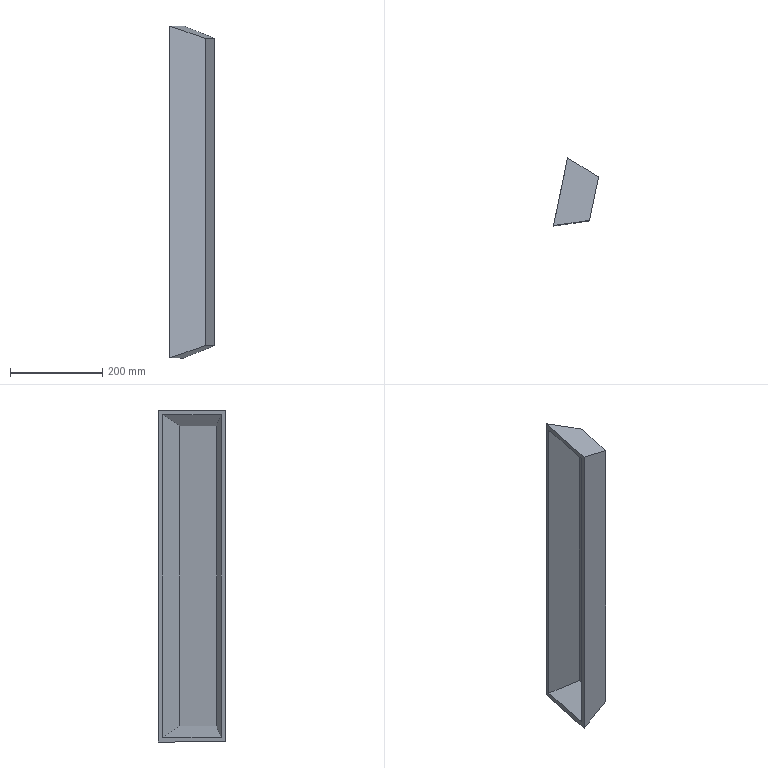Component | SolidWorks | AluminumIngotContainer-10 | 1 solid | 11 faces | box 97.54 x 146.85 x 720 mm | volume 1760907 mm3 | plane 11
build123d program:
from build123d import *

# Parameters (mm, degrees)
SKETCH1_W           = 150
SKETCH1_H           = 720
BOSS_EXTRUDE1_DEPTH = 74
BOSS_EXTRUDE1_TAPER = 20
SHELL1_T            = -10


with BuildPart() as part:
    # Sketch1 → Boss-Extrude1 (new body)
    with BuildSketch(Plane.XY):
        Rectangle(SKETCH1_W, SKETCH1_H)
    extrude(amount=BOSS_EXTRUDE1_DEPTH, taper=BOSS_EXTRUDE1_TAPER)

    # Shell1
    shell1_openings = [part.faces().sort_by_distance(p)[0] for p in [
        (0, 0, 0),
    ]]
    offset(amount=SHELL1_T, openings=shell1_openings, kind=Kind.INTERSECTION)


solid = part.part

# Placed as in the assembly
solid = solid.moved(Location((746.968, 361.921, 495), (90, 78.234, -180)))
STEP:
#1=COLOUR_RGB('',0.7922,0.8196,0.9333);
#2=FILL_AREA_STYLE_COLOUR('',#1);
#3=FILL_AREA_STYLE('',(#2));
#4=SURFACE_STYLE_FILL_AREA(#3);
#5=SURFACE_SIDE_STYLE('',(#4));
#6=SURFACE_STYLE_USAGE(.BOTH.,#5);
#7=PRESENTATION_STYLE_ASSIGNMENT((#6));
#8=CARTESIAN_POINT('',(30.01,17.14,5.315));
#9=VERTEX_POINT('',#8);
#10=CARTESIAN_POINT('',(30.01,17.14,33.661));
#11=VERTEX_POINT('',#10);
#12=CARTESIAN_POINT('',(30.01,17.14,5.315));
#13=DIRECTION('',(0.,0.,1.));
#14=VECTOR('',#13,39.37);
#15=LINE('',#12,#14);
#16=EDGE_CURVE('',#9,#11,#15,.T.);
#17=ORIENTED_EDGE('',*,*,#16,.F.);
#18=CARTESIAN_POINT('',(28.806,11.358,5.315));
#19=VERTEX_POINT('',#18);
#20=CARTESIAN_POINT('',(28.806,11.358,5.315));
#21=DIRECTION('',(0.2039,0.979,-0.));
#22=VECTOR('',#21,39.37);
#23=LINE('',#20,#22);
#24=EDGE_CURVE('',#19,#9,#23,.T.);
#25=ORIENTED_EDGE('',*,*,#24,.F.);
#26=CARTESIAN_POINT('',(28.806,11.358,33.661));
#27=VERTEX_POINT('',#26);
#28=CARTESIAN_POINT('',(28.806,11.358,5.315));
#29=DIRECTION('',(-0.,-0.,-1.));
#30=VECTOR('',#29,39.37);
#31=LINE('',#28,#30);
#32=EDGE_CURVE('',#27,#19,#31,.T.);
#33=ORIENTED_EDGE('',*,*,#32,.F.);
#34=CARTESIAN_POINT('',(28.806,11.358,33.661));
#35=DIRECTION('',(-0.2039,-0.979,0.));
#36=VECTOR('',#35,39.37);
#37=LINE('',#34,#36);
#38=EDGE_CURVE('',#11,#27,#37,.T.);
#39=ORIENTED_EDGE('',*,*,#38,.F.);
#40=EDGE_LOOP('',(#17,#25,#33,#39));
#41=FACE_OUTER_BOUND('',#40,.T.);
#42=CARTESIAN_POINT('',(28.892,11.768,5.734));
#43=VERTEX_POINT('',#42);
#44=CARTESIAN_POINT('',(29.925,16.729,5.734));
#45=VERTEX_POINT('',#44);
#46=CARTESIAN_POINT('',(29.408,14.249,5.734));
#47=DIRECTION('',(0.2039,0.979,-0.));
#48=VECTOR('',#47,39.37);
#49=LINE('',#46,#48);
#50=EDGE_CURVE('',#43,#45,#49,.T.);
#51=ORIENTED_EDGE('',*,*,#50,.T.);
#52=CARTESIAN_POINT('',(29.925,16.729,33.242));
#53=VERTEX_POINT('',#52);
#54=CARTESIAN_POINT('',(29.925,16.729,19.488));
#55=DIRECTION('',(0.,0.,1.));
#56=VECTOR('',#55,39.37);
#57=LINE('',#54,#56);
#58=EDGE_CURVE('',#45,#53,#57,.T.);
#59=ORIENTED_EDGE('',*,*,#58,.T.);
#60=CARTESIAN_POINT('',(28.892,11.768,33.242));
#61=VERTEX_POINT('',#60);
#62=CARTESIAN_POINT('',(29.408,14.249,33.242));
#63=DIRECTION('',(-0.2039,-0.979,0.));
#64=VECTOR('',#63,39.37);
#65=LINE('',#62,#64);
#66=EDGE_CURVE('',#53,#61,#65,.T.);
#67=ORIENTED_EDGE('',*,*,#66,.T.);
#68=CARTESIAN_POINT('',(28.892,11.768,19.488));
#69=DIRECTION('',(-0.,-0.,-1.));
#70=VECTOR('',#69,39.37);
#71=LINE('',#68,#70);
#72=EDGE_CURVE('',#61,#43,#71,.T.);
#73=ORIENTED_EDGE('',*,*,#72,.T.);
#74=EDGE_LOOP('',(#51,#59,#67,#73));
#75=FACE_BOUND('',#74,.T.);
#76=CARTESIAN_POINT('',(29.408,14.249,19.488));
#77=DIRECTION('',(-0.979,0.2039,0.));
#78=DIRECTION('',(0.2039,0.979,-0.));
#79=AXIS2_PLACEMENT_3D('',#76,#77,#78);
#80=PLANE('',#79);
#81=ADVANCED_FACE('',(#41,#75),#80,.T.);
#82=ORIENTED_EDGE('',*,*,#16,.T.);
#83=CARTESIAN_POINT('',(32.646,15.507,32.601));
#84=VERTEX_POINT('',#83);
#85=CARTESIAN_POINT('',(31.548,16.188,33.043));
#86=DIRECTION('',(-0.8045,0.4981,0.3236));
#87=VECTOR('',#86,39.37);
#88=LINE('',#85,#87);
#89=EDGE_CURVE('',#84,#11,#88,.T.);
#90=ORIENTED_EDGE('',*,*,#89,.F.);
#91=CARTESIAN_POINT('',(32.646,15.507,6.375));
#92=VERTEX_POINT('',#91);
#93=CARTESIAN_POINT('',(32.646,15.507,19.488));
#94=DIRECTION('',(0.,0.,1.));
#95=VECTOR('',#94,39.37);
#96=LINE('',#93,#95);
#97=EDGE_CURVE('',#92,#84,#96,.T.);
#98=ORIENTED_EDGE('',*,*,#97,.F.);
#99=CARTESIAN_POINT('',(30.01,17.14,5.315));
#100=DIRECTION('',(-0.8045,0.4981,-0.3236));
#101=VECTOR('',#100,39.37);
#102=LINE('',#99,#101);
#103=EDGE_CURVE('',#92,#9,#102,.T.);
#104=ORIENTED_EDGE('',*,*,#103,.T.);
#105=EDGE_LOOP('',(#82,#90,#98,#104));
#106=FACE_OUTER_BOUND('',#105,.T.);
#107=CARTESIAN_POINT('',(30.01,17.14,5.315));
#108=DIRECTION('',(0.5264,0.8502,-0.));
#109=DIRECTION('',(0.8502,-0.5264,-0.));
#110=AXIS2_PLACEMENT_3D('',#107,#108,#109);
#111=PLANE('',#110);
#112=ADVANCED_FACE('',(#106),#111,.T.);
#113=ORIENTED_EDGE('',*,*,#38,.T.);
#114=CARTESIAN_POINT('',(31.874,11.802,32.601));
#115=VERTEX_POINT('',#114);
#116=CARTESIAN_POINT('',(37.396,12.601,30.693));
#117=DIRECTION('',(-0.9364,-0.1355,0.3236));
#118=VECTOR('',#117,39.37);
#119=LINE('',#116,#118);
#120=EDGE_CURVE('',#115,#27,#119,.T.);
#121=ORIENTED_EDGE('',*,*,#120,.F.);
#122=CARTESIAN_POINT('',(32.26,13.655,32.601));
#123=DIRECTION('',(-0.2039,-0.979,0.));
#124=VECTOR('',#123,39.37);
#125=LINE('',#122,#124);
#126=EDGE_CURVE('',#84,#115,#125,.T.);
#127=ORIENTED_EDGE('',*,*,#126,.F.);
#128=ORIENTED_EDGE('',*,*,#89,.T.);
#129=EDGE_LOOP('',(#113,#121,#127,#128));
#130=FACE_OUTER_BOUND('',#129,.T.);
#131=CARTESIAN_POINT('',(28.806,11.358,33.661));
#132=DIRECTION('',(0.3348,-0.06974,0.9397));
#133=DIRECTION('',(-0.9199,0.1916,0.342));
#134=AXIS2_PLACEMENT_3D('',#131,#132,#133);
#135=PLANE('',#134);
#136=ADVANCED_FACE('',(#130),#135,.T.);
#137=ORIENTED_EDGE('',*,*,#32,.T.);
#138=CARTESIAN_POINT('',(31.874,11.802,6.375));
#139=VERTEX_POINT('',#138);
#140=CARTESIAN_POINT('',(28.806,11.358,5.315));
#141=DIRECTION('',(-0.9364,-0.1355,-0.3236));
#142=VECTOR('',#141,39.37);
#143=LINE('',#140,#142);
#144=EDGE_CURVE('',#139,#19,#143,.T.);
#145=ORIENTED_EDGE('',*,*,#144,.F.);
#146=CARTESIAN_POINT('',(31.874,11.802,19.488));
#147=DIRECTION('',(-0.,-0.,-1.));
#148=VECTOR('',#147,39.37);
#149=LINE('',#146,#148);
#150=EDGE_CURVE('',#115,#139,#149,.T.);
#151=ORIENTED_EDGE('',*,*,#150,.F.);
#152=ORIENTED_EDGE('',*,*,#120,.T.);
#153=EDGE_LOOP('',(#137,#145,#151,#152));
#154=FACE_OUTER_BOUND('',#153,.T.);
#155=CARTESIAN_POINT('',(28.806,11.358,5.315));
#156=DIRECTION('',(0.1432,-0.9897,0.));
#157=DIRECTION('',(-0.9897,-0.1432,0.));
#158=AXIS2_PLACEMENT_3D('',#155,#156,#157);
#159=PLANE('',#158);
#160=ADVANCED_FACE('',(#154),#159,.T.);
#161=ORIENTED_EDGE('',*,*,#24,.T.);
#162=ORIENTED_EDGE('',*,*,#103,.F.);
#163=CARTESIAN_POINT('',(32.26,13.655,6.375));
#164=DIRECTION('',(0.2039,0.979,-0.));
#165=VECTOR('',#164,39.37);
#166=LINE('',#163,#165);
#167=EDGE_CURVE('',#139,#92,#166,.T.);
#168=ORIENTED_EDGE('',*,*,#167,.F.);
#169=ORIENTED_EDGE('',*,*,#144,.T.);
#170=EDGE_LOOP('',(#161,#162,#168,#169));
#171=FACE_OUTER_BOUND('',#170,.T.);
#172=CARTESIAN_POINT('',(28.806,11.358,5.315));
#173=DIRECTION('',(0.3348,-0.06974,-0.9397));
#174=DIRECTION('',(0.9199,-0.1916,0.342));
#175=AXIS2_PLACEMENT_3D('',#172,#173,#174);
#176=PLANE('',#175);
#177=ADVANCED_FACE('',(#171),#176,.T.);
#178=ORIENTED_EDGE('',*,*,#97,.T.);
#179=ORIENTED_EDGE('',*,*,#126,.T.);
#180=ORIENTED_EDGE('',*,*,#150,.T.);
#181=ORIENTED_EDGE('',*,*,#167,.T.);
#182=EDGE_LOOP('',(#178,#179,#180,#181));
#183=FACE_OUTER_BOUND('',#182,.T.);
#184=CARTESIAN_POINT('',(32.26,13.655,19.488));
#185=DIRECTION('',(-0.979,0.2039,0.));
#186=DIRECTION('',(0.2039,0.979,-0.));
#187=AXIS2_PLACEMENT_3D('',#184,#185,#186);
#188=PLANE('',#187);
#189=ADVANCED_FACE('',(#183),#188,.F.);
#190=ORIENTED_EDGE('',*,*,#58,.F.);
#191=CARTESIAN_POINT('',(32.205,15.318,6.651));
#192=VERTEX_POINT('',#191);
#193=CARTESIAN_POINT('',(29.707,16.864,5.646));
#194=DIRECTION('',(-0.8045,0.4981,-0.3236));
#195=VECTOR('',#194,39.37);
#196=LINE('',#193,#195);
#197=EDGE_CURVE('',#192,#45,#196,.T.);
#198=ORIENTED_EDGE('',*,*,#197,.F.);
#199=CARTESIAN_POINT('',(32.205,15.318,32.325));
#200=VERTEX_POINT('',#199);
#201=CARTESIAN_POINT('',(32.205,15.318,19.488));
#202=DIRECTION('',(0.,0.,1.));
#203=VECTOR('',#202,39.37);
#204=LINE('',#201,#203);
#205=EDGE_CURVE('',#192,#200,#204,.T.);
#206=ORIENTED_EDGE('',*,*,#205,.T.);
#207=CARTESIAN_POINT('',(31.244,15.913,32.712));
#208=DIRECTION('',(-0.8045,0.4981,0.3236));
#209=VECTOR('',#208,39.37);
#210=LINE('',#207,#209);
#211=EDGE_CURVE('',#200,#53,#210,.T.);
#212=ORIENTED_EDGE('',*,*,#211,.T.);
#213=EDGE_LOOP('',(#190,#198,#206,#212));
#214=FACE_OUTER_BOUND('',#213,.T.);
#215=CARTESIAN_POINT('',(29.803,16.805,5.315));
#216=DIRECTION('',(0.5264,0.8502,-0.));
#217=DIRECTION('',(0.8502,-0.5264,-0.));
#218=AXIS2_PLACEMENT_3D('',#215,#216,#217);
#219=PLANE('',#218);
#220=ADVANCED_FACE('',(#214),#219,.F.);
#221=ORIENTED_EDGE('',*,*,#66,.F.);
#222=ORIENTED_EDGE('',*,*,#211,.F.);
#223=CARTESIAN_POINT('',(31.545,12.152,32.325));
#224=VERTEX_POINT('',#223);
#225=CARTESIAN_POINT('',(31.875,13.735,32.325));
#226=DIRECTION('',(-0.2039,-0.979,0.));
#227=VECTOR('',#226,39.37);
#228=LINE('',#225,#227);
#229=EDGE_CURVE('',#200,#224,#228,.T.);
#230=ORIENTED_EDGE('',*,*,#229,.T.);
#231=CARTESIAN_POINT('',(37.228,12.975,30.362));
#232=DIRECTION('',(-0.9364,-0.1355,0.3236));
#233=VECTOR('',#232,39.37);
#234=LINE('',#231,#233);
#235=EDGE_CURVE('',#224,#61,#234,.T.);
#236=ORIENTED_EDGE('',*,*,#235,.T.);
#237=EDGE_LOOP('',(#221,#222,#230,#236));
#238=FACE_OUTER_BOUND('',#237,.T.);
#239=CARTESIAN_POINT('',(28.674,11.386,33.291));
#240=DIRECTION('',(0.3348,-0.06974,0.9397));
#241=DIRECTION('',(-0.9199,0.1916,0.342));
#242=AXIS2_PLACEMENT_3D('',#239,#240,#241);
#243=PLANE('',#242);
#244=ADVANCED_FACE('',(#238),#243,.F.);
#245=ORIENTED_EDGE('',*,*,#72,.F.);
#246=ORIENTED_EDGE('',*,*,#235,.F.);
#247=CARTESIAN_POINT('',(31.545,12.152,6.651));
#248=VERTEX_POINT('',#247);
#249=CARTESIAN_POINT('',(31.545,12.152,19.488));
#250=DIRECTION('',(-0.,-0.,-1.));
#251=VECTOR('',#250,39.37);
#252=LINE('',#249,#251);
#253=EDGE_CURVE('',#224,#248,#252,.T.);
#254=ORIENTED_EDGE('',*,*,#253,.T.);
#255=CARTESIAN_POINT('',(28.638,11.732,5.646));
#256=DIRECTION('',(-0.9364,-0.1355,-0.3236));
#257=VECTOR('',#256,39.37);
#258=LINE('',#255,#257);
#259=EDGE_CURVE('',#248,#43,#258,.T.);
#260=ORIENTED_EDGE('',*,*,#259,.T.);
#261=EDGE_LOOP('',(#245,#246,#254,#260));
#262=FACE_OUTER_BOUND('',#261,.T.);
#263=CARTESIAN_POINT('',(28.75,11.748,5.315));
#264=DIRECTION('',(0.1432,-0.9897,0.));
#265=DIRECTION('',(-0.9897,-0.1432,0.));
#266=AXIS2_PLACEMENT_3D('',#263,#264,#265);
#267=PLANE('',#266);
#268=ADVANCED_FACE('',(#262),#267,.F.);
#269=ORIENTED_EDGE('',*,*,#50,.F.);
#270=ORIENTED_EDGE('',*,*,#259,.F.);
#271=CARTESIAN_POINT('',(31.875,13.735,6.651));
#272=DIRECTION('',(0.2039,0.979,-0.));
#273=VECTOR('',#272,39.37);
#274=LINE('',#271,#273);
#275=EDGE_CURVE('',#248,#192,#274,.T.);
#276=ORIENTED_EDGE('',*,*,#275,.T.);
#277=ORIENTED_EDGE('',*,*,#197,.T.);
#278=EDGE_LOOP('',(#269,#270,#276,#277));
#279=FACE_OUTER_BOUND('',#278,.T.);
#280=CARTESIAN_POINT('',(28.674,11.386,5.685));
#281=DIRECTION('',(0.3348,-0.06974,-0.9397));
#282=DIRECTION('',(0.9199,-0.1916,0.342));
#283=AXIS2_PLACEMENT_3D('',#280,#281,#282);
#284=PLANE('',#283);
#285=ADVANCED_FACE('',(#279),#284,.F.);
#286=ORIENTED_EDGE('',*,*,#205,.F.);
#287=ORIENTED_EDGE('',*,*,#275,.F.);
#288=ORIENTED_EDGE('',*,*,#253,.F.);
#289=ORIENTED_EDGE('',*,*,#229,.F.);
#290=EDGE_LOOP('',(#286,#287,#288,#289));
#291=FACE_OUTER_BOUND('',#290,.T.);
#292=CARTESIAN_POINT('',(31.875,13.735,19.488));
#293=DIRECTION('',(-0.979,0.2039,0.));
#294=DIRECTION('',(0.2039,0.979,-0.));
#295=AXIS2_PLACEMENT_3D('',#292,#293,#294);
#296=PLANE('',#295);
#297=ADVANCED_FACE('',(#291),#296,.T.);
#298=CLOSED_SHELL('',(#81,#112,#136,#160,#177,#189,#220,#244,#268,#285,#297));
#299=MANIFOLD_SOLID_BREP('',#298);
#300=STYLED_ITEM('',(#7),#299);
#301=(LENGTH_UNIT()NAMED_UNIT(*)SI_UNIT($,.METRE.));
#302=LENGTH_MEASURE_WITH_UNIT(LENGTH_MEASURE(0.0254),#301);
#303=DIMENSIONAL_EXPONENTS(1.,0.,0.,0.,0.,0.,0.);
#304=(CONVERSION_BASED_UNIT('',#302)LENGTH_UNIT()NAMED_UNIT(#303));
#305=UNCERTAINTY_MEASURE_WITH_UNIT(LENGTH_MEASURE(0.00001),#304,'','');
#306=(NAMED_UNIT(*)PLANE_ANGLE_UNIT()SI_UNIT($,.RADIAN.));
#307=(NAMED_UNIT(*)SI_UNIT($,.STERADIAN.)SOLID_ANGLE_UNIT());
#308=(GEOMETRIC_REPRESENTATION_CONTEXT(3)GLOBAL_UNCERTAINTY_ASSIGNED_CONTEXT((#305))GLOBAL_UNIT_ASSIGNED_CONTEXT((#304,#306,#307))REPRESENTATION_CONTEXT('',''));
#309=MECHANICAL_DESIGN_GEOMETRIC_PRESENTATION_REPRESENTATION('',(#300),#308);
#310=PRESENTATION_LAYER_ASSIGNMENT('','',(#300));
#311=CARTESIAN_POINT('',(0.,0.,0.));
#312=DIRECTION('',(0.,0.,1.));
#313=DIRECTION('',(1.,0.,0.));
#314=AXIS2_PLACEMENT_3D('',#311,#312,#313);
#315=(LENGTH_UNIT()NAMED_UNIT(*)SI_UNIT($,.METRE.));
#316=LENGTH_MEASURE_WITH_UNIT(LENGTH_MEASURE(0.0254),#315);
#317=DIMENSIONAL_EXPONENTS(1.,0.,0.,0.,0.,0.,0.);
#318=(CONVERSION_BASED_UNIT('',#316)LENGTH_UNIT()NAMED_UNIT(#317));
#319=UNCERTAINTY_MEASURE_WITH_UNIT(LENGTH_MEASURE(0.00001),#318,'','');
#320=(NAMED_UNIT(*)PLANE_ANGLE_UNIT()SI_UNIT($,.RADIAN.));
#321=(NAMED_UNIT(*)SI_UNIT($,.STERADIAN.)SOLID_ANGLE_UNIT());
#322=(GEOMETRIC_REPRESENTATION_CONTEXT(3)GLOBAL_UNCERTAINTY_ASSIGNED_CONTEXT((#319))GLOBAL_UNIT_ASSIGNED_CONTEXT((#318,#320,#321))REPRESENTATION_CONTEXT('',''));
#323=ADVANCED_BREP_SHAPE_REPRESENTATION('',(#299,#314),#322);